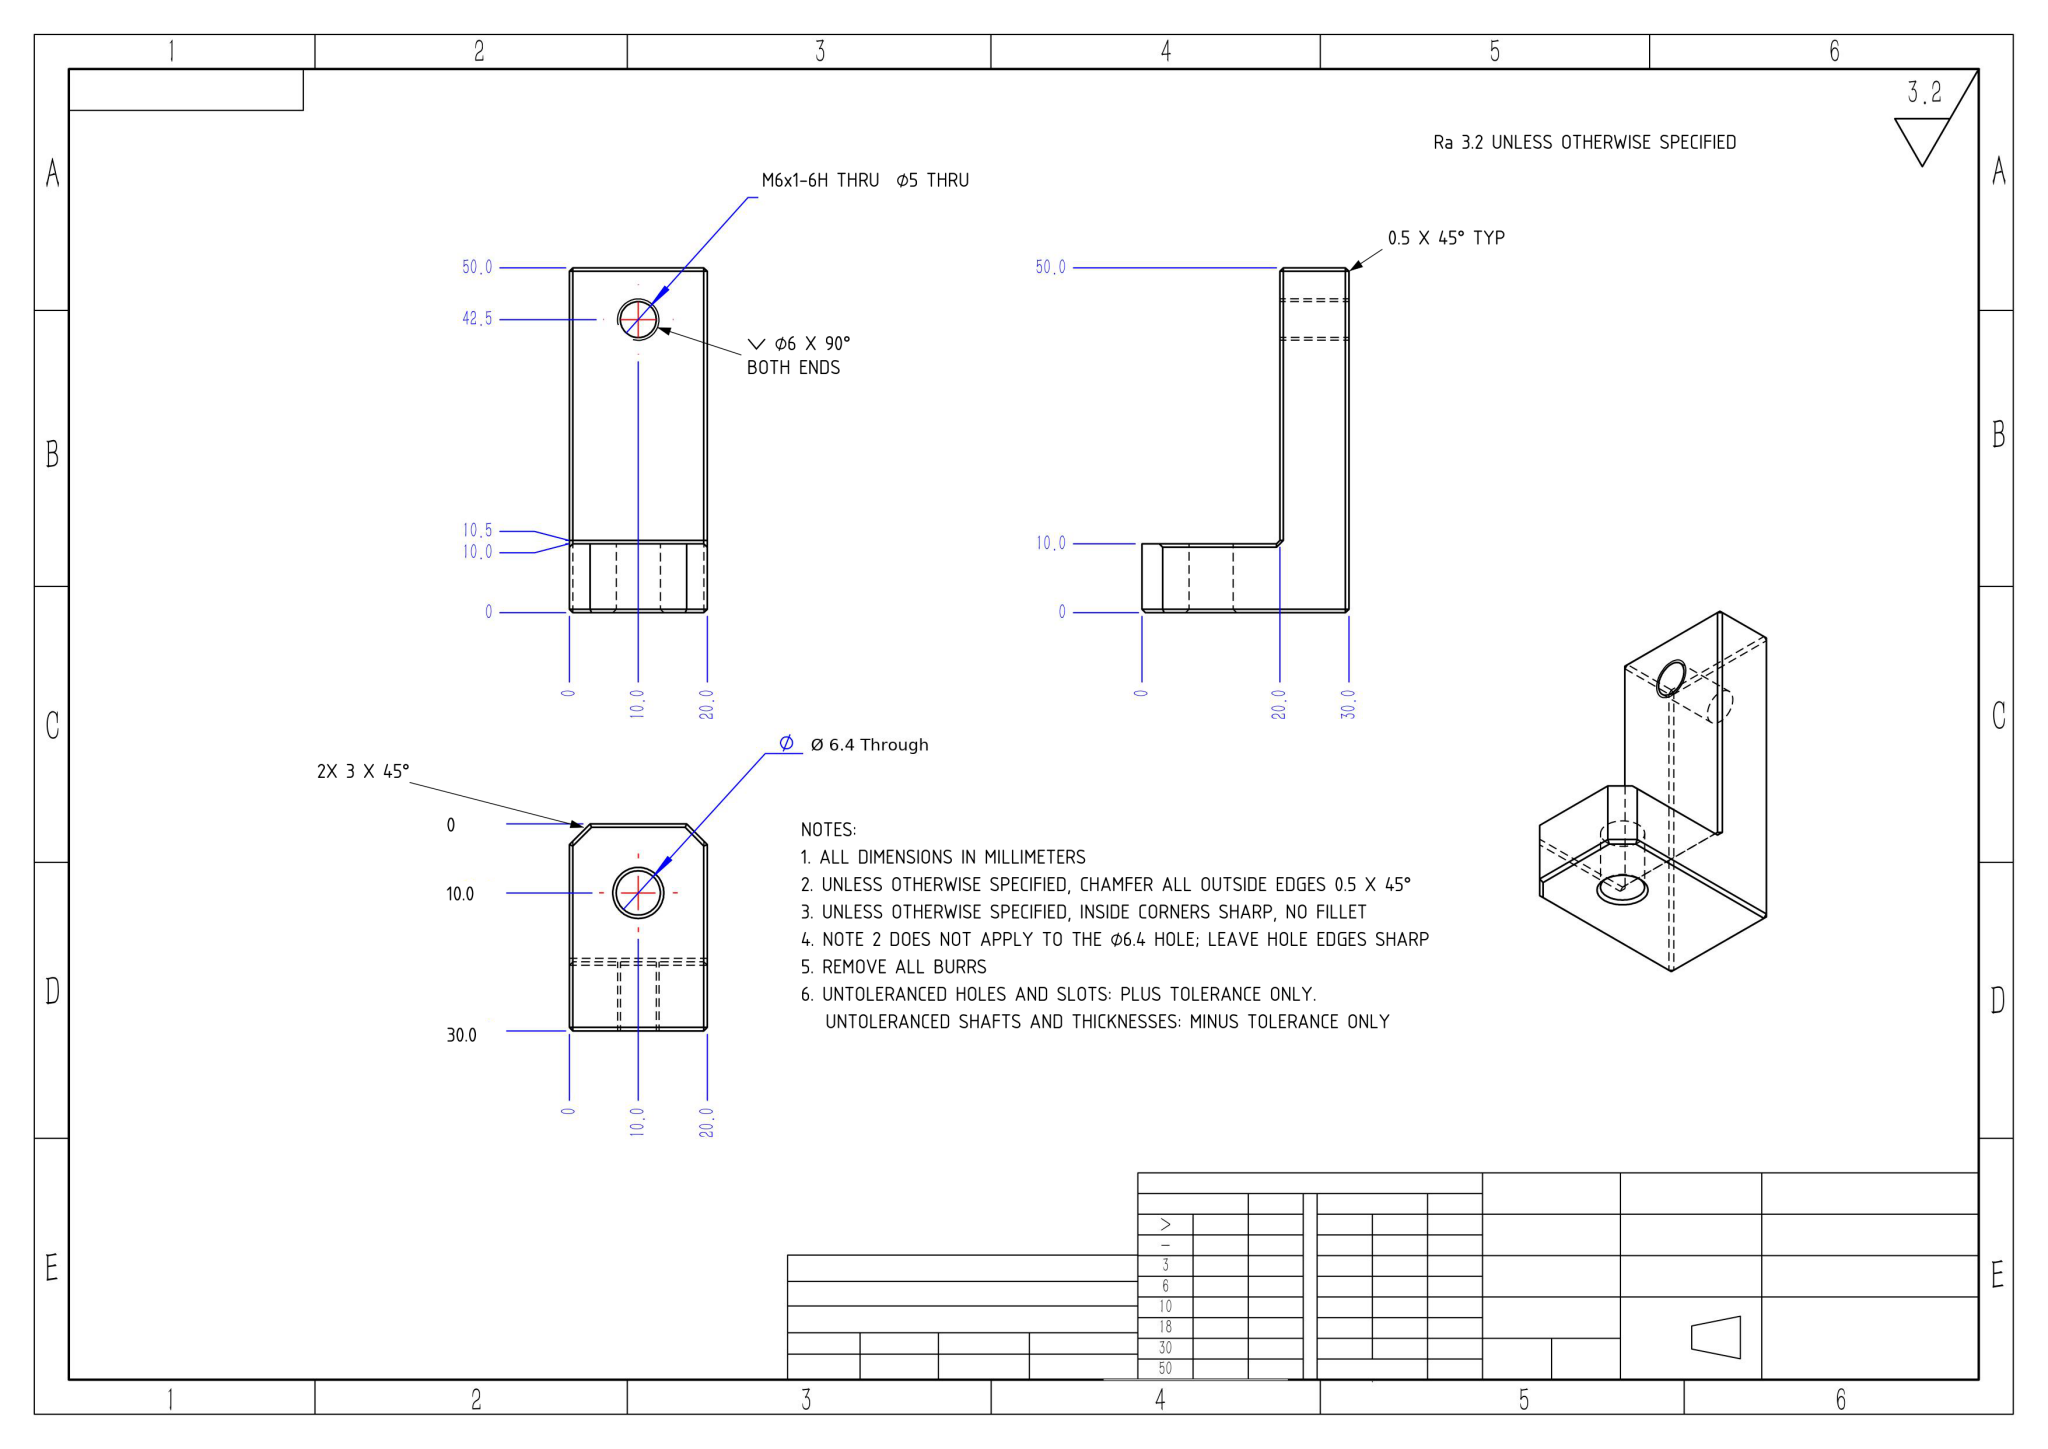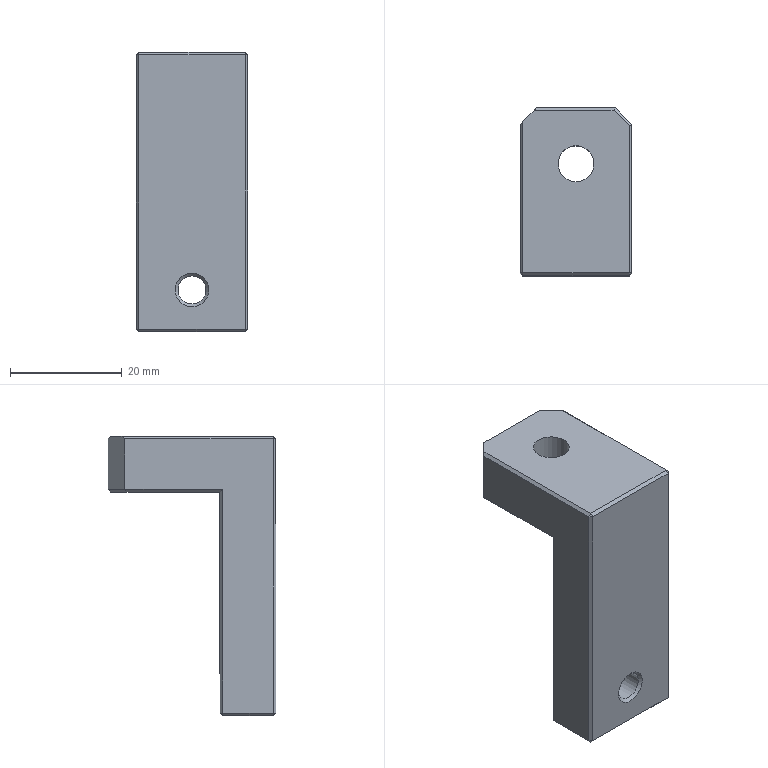Part | NX | mm | 1 solid | 38 faces | box 20.01 x 30.01 x 50 mm | volume 13340 mm3 | plane 34 | cylinder 2 | cone 2 | commonest cylinder face diameters 6.4 x1 5 x1